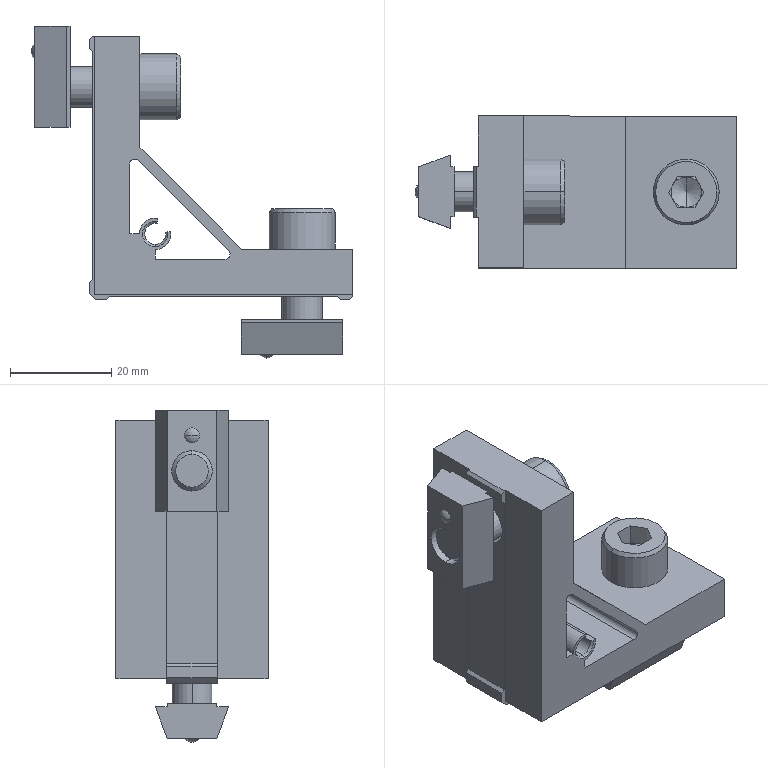Component | SolidWorks | Q1-A12-S21-Q1B.SLDASQ-1_Q1-HBKTS8-C-SEP-1 | 5 solids | 136 faces | volume 31127 mm3 | plane 83 | cylinder 27 | cone 18 | sphere 4 | torus 4 | commonest cylinder face diameters 8 x8 9 x4 13 x4 4.134 x3 6.2 x3 2 x3 3 x2 | material 6061